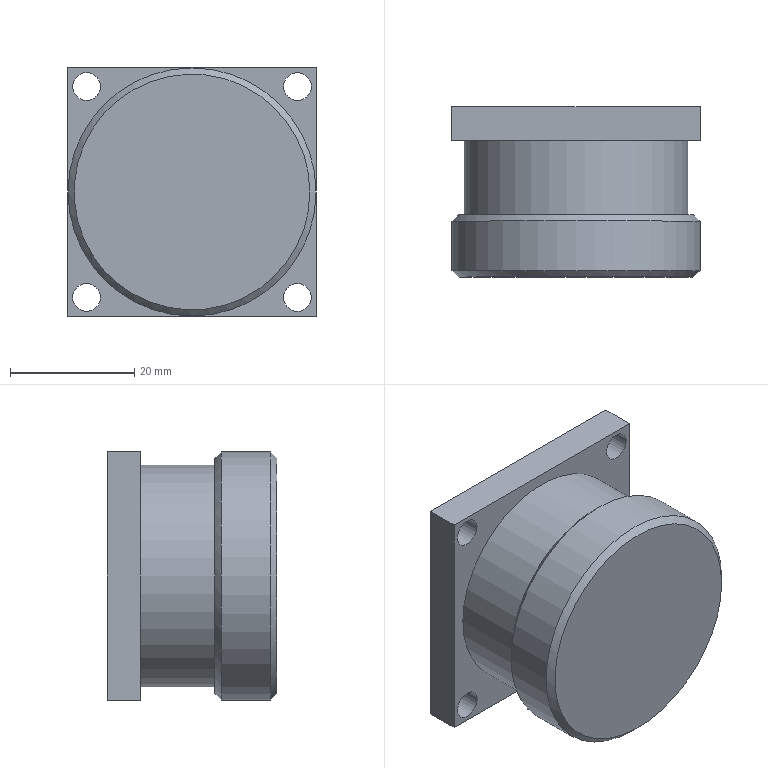Component | NX | BUTTON | 1 solid | 16 faces | box 40 x 27.4 x 40 mm | volume 32954 mm3 | plane 8 | cylinder 6 | cone 2 | commonest cylinder face diameters 4.5 x4 36 x1 40 x1
STEP:
#1=CARTESIAN_POINT('',(0.,0.,0.));
#2=DIRECTION('',(0.,0.,1.));
#3=DIRECTION('',(1.,0.,0.));
#4=AXIS2_PLACEMENT_3D('',#1,#2,#3);
#5=CARTESIAN_POINT('',(-20.,-310.4,-247.));
#6=VERTEX_POINT('',#5);
#7=CARTESIAN_POINT('',(-20.,-310.4,-287.));
#8=VERTEX_POINT('',#7);
#9=CARTESIAN_POINT('',(-20.,-310.4,-247.));
#10=DIRECTION('',(0.,0.,-1.));
#11=VECTOR('',#10,1.);
#12=LINE('',#9,#11);
#13=CARTESIAN_POINT('',(-20.,-305.,-247.));
#14=DIRECTION('',(-1.,0.,0.));
#15=DIRECTION('',(0.,-1.,0.));
#16=AXIS2_PLACEMENT_3D('',#13,#14,#15);
#17=PLANE('',#16);
#18=CARTESIAN_POINT('',(5.4,0.));
#19=DIRECTION('',(0.,-1.));
#20=VECTOR('',#19,1.);
#21=LINE('',#18,#20);
#22=(GEOMETRIC_REPRESENTATION_CONTEXT(2)PARAMETRIC_REPRESENTATION_CONTEXT()REPRESENTATION_CONTEXT('',''));
#23=DEFINITIONAL_REPRESENTATION('',(#21),#22);
#24=PCURVE('',#17,#23);
#25=CARTESIAN_POINT('',(-17.,-310.4,-284.));
#26=DIRECTION('',(0.,-1.,0.));
#27=DIRECTION('',(1.,0.,0.));
#28=AXIS2_PLACEMENT_3D('',#25,#26,#27);
#29=PLANE('',#28);
#30=CARTESIAN_POINT('',(-3.,37.));
#31=DIRECTION('',(0.,-1.));
#32=VECTOR('',#31,1.);
#33=LINE('',#30,#32);
#34=(GEOMETRIC_REPRESENTATION_CONTEXT(2)PARAMETRIC_REPRESENTATION_CONTEXT()REPRESENTATION_CONTEXT('',''));
#35=DEFINITIONAL_REPRESENTATION('',(#33),#34);
#36=PCURVE('',#29,#35);
#37=SURFACE_CURVE('',#12,(#24,#36),.PCURVE_S1.);
#38=EDGE_CURVE('',#6,#8,#37,.T.);
#39=ORIENTED_EDGE('',*,*,#38,.F.);
#40=CARTESIAN_POINT('',(-20.,-305.,-247.));
#41=VERTEX_POINT('',#40);
#42=CARTESIAN_POINT('',(-20.,-305.,-247.));
#43=DIRECTION('',(0.,-1.,0.));
#44=VECTOR('',#43,1.);
#45=LINE('',#42,#44);
#46=CARTESIAN_POINT('',(0.,0.));
#47=DIRECTION('',(1.,0.));
#48=VECTOR('',#47,1.);
#49=LINE('',#46,#48);
#50=(GEOMETRIC_REPRESENTATION_CONTEXT(2)PARAMETRIC_REPRESENTATION_CONTEXT()REPRESENTATION_CONTEXT('',''));
#51=DEFINITIONAL_REPRESENTATION('',(#49),#50);
#52=PCURVE('',#17,#51);
#53=CARTESIAN_POINT('',(20.,-305.,-247.));
#54=DIRECTION('',(0.,0.,1.));
#55=DIRECTION('',(0.,-1.,0.));
#56=AXIS2_PLACEMENT_3D('',#53,#54,#55);
#57=PLANE('',#56);
#58=CARTESIAN_POINT('',(0.,-40.));
#59=DIRECTION('',(1.,0.));
#60=VECTOR('',#59,1.);
#61=LINE('',#58,#60);
#62=(GEOMETRIC_REPRESENTATION_CONTEXT(2)PARAMETRIC_REPRESENTATION_CONTEXT()REPRESENTATION_CONTEXT('',''));
#63=DEFINITIONAL_REPRESENTATION('',(#61),#62);
#64=PCURVE('',#57,#63);
#65=SURFACE_CURVE('',#45,(#52,#64),.PCURVE_S1.);
#66=EDGE_CURVE('',#41,#6,#65,.T.);
#67=ORIENTED_EDGE('',*,*,#66,.F.);
#68=CARTESIAN_POINT('',(-20.,-305.,-287.));
#69=VERTEX_POINT('',#68);
#70=CARTESIAN_POINT('',(-20.,-305.,-247.));
#71=DIRECTION('',(0.,0.,-1.));
#72=VECTOR('',#71,1.);
#73=LINE('',#70,#72);
#74=CARTESIAN_POINT('',(0.,0.));
#75=DIRECTION('',(0.,-1.));
#76=VECTOR('',#75,1.);
#77=LINE('',#74,#76);
#78=(GEOMETRIC_REPRESENTATION_CONTEXT(2)PARAMETRIC_REPRESENTATION_CONTEXT()REPRESENTATION_CONTEXT('',''));
#79=DEFINITIONAL_REPRESENTATION('',(#77),#78);
#80=PCURVE('',#17,#79);
#81=CARTESIAN_POINT('',(-17.,-305.,-284.));
#82=DIRECTION('',(0.,-1.,0.));
#83=DIRECTION('',(1.,0.,0.));
#84=AXIS2_PLACEMENT_3D('',#81,#82,#83);
#85=PLANE('',#84);
#86=CARTESIAN_POINT('',(-3.,37.));
#87=DIRECTION('',(0.,-1.));
#88=VECTOR('',#87,1.);
#89=LINE('',#86,#88);
#90=(GEOMETRIC_REPRESENTATION_CONTEXT(2)PARAMETRIC_REPRESENTATION_CONTEXT()REPRESENTATION_CONTEXT('',''));
#91=DEFINITIONAL_REPRESENTATION('',(#89),#90);
#92=PCURVE('',#85,#91);
#93=SURFACE_CURVE('',#73,(#80,#92),.PCURVE_S1.);
#94=EDGE_CURVE('',#41,#69,#93,.T.);
#95=ORIENTED_EDGE('',*,*,#94,.T.);
#96=CARTESIAN_POINT('',(-20.,-305.,-287.));
#97=DIRECTION('',(0.,-1.,0.));
#98=VECTOR('',#97,1.);
#99=LINE('',#96,#98);
#100=CARTESIAN_POINT('',(0.,-40.));
#101=DIRECTION('',(1.,0.));
#102=VECTOR('',#101,1.);
#103=LINE('',#100,#102);
#104=(GEOMETRIC_REPRESENTATION_CONTEXT(2)PARAMETRIC_REPRESENTATION_CONTEXT()REPRESENTATION_CONTEXT('',''));
#105=DEFINITIONAL_REPRESENTATION('',(#103),#104);
#106=PCURVE('',#17,#105);
#107=CARTESIAN_POINT('',(-20.,-305.,-287.));
#108=DIRECTION('',(0.,0.,-1.));
#109=DIRECTION('',(0.,1.,0.));
#110=AXIS2_PLACEMENT_3D('',#107,#108,#109);
#111=PLANE('',#110);
#112=CARTESIAN_POINT('',(0.,0.));
#113=DIRECTION('',(-1.,0.));
#114=VECTOR('',#113,1.);
#115=LINE('',#112,#114);
#116=(GEOMETRIC_REPRESENTATION_CONTEXT(2)PARAMETRIC_REPRESENTATION_CONTEXT()REPRESENTATION_CONTEXT('',''));
#117=DEFINITIONAL_REPRESENTATION('',(#115),#116);
#118=PCURVE('',#111,#117);
#119=SURFACE_CURVE('',#99,(#106,#118),.PCURVE_S1.);
#120=EDGE_CURVE('',#69,#8,#119,.T.);
#121=ORIENTED_EDGE('',*,*,#120,.T.);
#122=EDGE_LOOP('',(#39,#67,#95,#121));
#123=FACE_BOUND('',#122,.T.);
#124=ADVANCED_FACE('',(#123),#17,.T.);
#125=CARTESIAN_POINT('',(20.,-310.4,-287.));
#126=VERTEX_POINT('',#125);
#127=CARTESIAN_POINT('',(-20.,-310.4,-287.));
#128=DIRECTION('',(1.,0.,0.));
#129=VECTOR('',#128,1.);
#130=LINE('',#127,#129);
#131=CARTESIAN_POINT('',(-5.4,0.));
#132=DIRECTION('',(0.,1.));
#133=VECTOR('',#132,1.);
#134=LINE('',#131,#133);
#135=(GEOMETRIC_REPRESENTATION_CONTEXT(2)PARAMETRIC_REPRESENTATION_CONTEXT()REPRESENTATION_CONTEXT('',''));
#136=DEFINITIONAL_REPRESENTATION('',(#134),#135);
#137=PCURVE('',#111,#136);
#138=CARTESIAN_POINT('',(-3.,-3.));
#139=DIRECTION('',(1.,0.));
#140=VECTOR('',#139,1.);
#141=LINE('',#138,#140);
#142=(GEOMETRIC_REPRESENTATION_CONTEXT(2)PARAMETRIC_REPRESENTATION_CONTEXT()REPRESENTATION_CONTEXT('',''));
#143=DEFINITIONAL_REPRESENTATION('',(#141),#142);
#144=PCURVE('',#29,#143);
#145=SURFACE_CURVE('',#130,(#137,#144),.PCURVE_S1.);
#146=EDGE_CURVE('',#8,#126,#145,.T.);
#147=ORIENTED_EDGE('',*,*,#146,.F.);
#148=ORIENTED_EDGE('',*,*,#120,.F.);
#149=CARTESIAN_POINT('',(20.,-305.,-287.));
#150=VERTEX_POINT('',#149);
#151=CARTESIAN_POINT('',(-20.,-305.,-287.));
#152=DIRECTION('',(1.,0.,0.));
#153=VECTOR('',#152,1.);
#154=LINE('',#151,#153);
#155=CARTESIAN_POINT('',(0.,0.));
#156=DIRECTION('',(0.,1.));
#157=VECTOR('',#156,1.);
#158=LINE('',#155,#157);
#159=(GEOMETRIC_REPRESENTATION_CONTEXT(2)PARAMETRIC_REPRESENTATION_CONTEXT()REPRESENTATION_CONTEXT('',''));
#160=DEFINITIONAL_REPRESENTATION('',(#158),#159);
#161=PCURVE('',#111,#160);
#162=CARTESIAN_POINT('',(-3.,-3.));
#163=DIRECTION('',(1.,0.));
#164=VECTOR('',#163,1.);
#165=LINE('',#162,#164);
#166=(GEOMETRIC_REPRESENTATION_CONTEXT(2)PARAMETRIC_REPRESENTATION_CONTEXT()REPRESENTATION_CONTEXT('',''));
#167=DEFINITIONAL_REPRESENTATION('',(#165),#166);
#168=PCURVE('',#85,#167);
#169=SURFACE_CURVE('',#154,(#161,#168),.PCURVE_S1.);
#170=EDGE_CURVE('',#69,#150,#169,.T.);
#171=ORIENTED_EDGE('',*,*,#170,.T.);
#172=CARTESIAN_POINT('',(20.,-305.,-287.));
#173=DIRECTION('',(0.,-1.,0.));
#174=VECTOR('',#173,1.);
#175=LINE('',#172,#174);
#176=CARTESIAN_POINT('',(0.,40.));
#177=DIRECTION('',(-1.,0.));
#178=VECTOR('',#177,1.);
#179=LINE('',#176,#178);
#180=(GEOMETRIC_REPRESENTATION_CONTEXT(2)PARAMETRIC_REPRESENTATION_CONTEXT()REPRESENTATION_CONTEXT('',''));
#181=DEFINITIONAL_REPRESENTATION('',(#179),#180);
#182=PCURVE('',#111,#181);
#183=CARTESIAN_POINT('',(20.,-305.,-287.));
#184=DIRECTION('',(1.,0.,0.));
#185=DIRECTION('',(0.,1.,0.));
#186=AXIS2_PLACEMENT_3D('',#183,#184,#185);
#187=PLANE('',#186);
#188=CARTESIAN_POINT('',(0.,0.));
#189=DIRECTION('',(-1.,0.));
#190=VECTOR('',#189,1.);
#191=LINE('',#188,#190);
#192=(GEOMETRIC_REPRESENTATION_CONTEXT(2)PARAMETRIC_REPRESENTATION_CONTEXT()REPRESENTATION_CONTEXT('',''));
#193=DEFINITIONAL_REPRESENTATION('',(#191),#192);
#194=PCURVE('',#187,#193);
#195=SURFACE_CURVE('',#175,(#182,#194),.PCURVE_S1.);
#196=EDGE_CURVE('',#150,#126,#195,.T.);
#197=ORIENTED_EDGE('',*,*,#196,.T.);
#198=EDGE_LOOP('',(#147,#148,#171,#197));
#199=FACE_BOUND('',#198,.T.);
#200=ADVANCED_FACE('',(#199),#111,.T.);
#201=CARTESIAN_POINT('',(20.,-310.4,-247.));
#202=VERTEX_POINT('',#201);
#203=CARTESIAN_POINT('',(20.,-310.4,-287.));
#204=DIRECTION('',(0.,0.,1.));
#205=VECTOR('',#204,1.);
#206=LINE('',#203,#205);
#207=CARTESIAN_POINT('',(-5.4,0.));
#208=DIRECTION('',(0.,1.));
#209=VECTOR('',#208,1.);
#210=LINE('',#207,#209);
#211=(GEOMETRIC_REPRESENTATION_CONTEXT(2)PARAMETRIC_REPRESENTATION_CONTEXT()REPRESENTATION_CONTEXT('',''));
#212=DEFINITIONAL_REPRESENTATION('',(#210),#211);
#213=PCURVE('',#187,#212);
#214=CARTESIAN_POINT('',(37.,-3.));
#215=DIRECTION('',(0.,1.));
#216=VECTOR('',#215,1.);
#217=LINE('',#214,#216);
#218=(GEOMETRIC_REPRESENTATION_CONTEXT(2)PARAMETRIC_REPRESENTATION_CONTEXT()REPRESENTATION_CONTEXT('',''));
#219=DEFINITIONAL_REPRESENTATION('',(#217),#218);
#220=PCURVE('',#29,#219);
#221=SURFACE_CURVE('',#206,(#213,#220),.PCURVE_S1.);
#222=EDGE_CURVE('',#126,#202,#221,.T.);
#223=ORIENTED_EDGE('',*,*,#222,.F.);
#224=ORIENTED_EDGE('',*,*,#196,.F.);
#225=CARTESIAN_POINT('',(20.,-305.,-247.));
#226=VERTEX_POINT('',#225);
#227=CARTESIAN_POINT('',(20.,-305.,-287.));
#228=DIRECTION('',(0.,0.,1.));
#229=VECTOR('',#228,1.);
#230=LINE('',#227,#229);
#231=CARTESIAN_POINT('',(0.,0.));
#232=DIRECTION('',(0.,1.));
#233=VECTOR('',#232,1.);
#234=LINE('',#231,#233);
#235=(GEOMETRIC_REPRESENTATION_CONTEXT(2)PARAMETRIC_REPRESENTATION_CONTEXT()REPRESENTATION_CONTEXT('',''));
#236=DEFINITIONAL_REPRESENTATION('',(#234),#235);
#237=PCURVE('',#187,#236);
#238=CARTESIAN_POINT('',(37.,-3.));
#239=DIRECTION('',(0.,1.));
#240=VECTOR('',#239,1.);
#241=LINE('',#238,#240);
#242=(GEOMETRIC_REPRESENTATION_CONTEXT(2)PARAMETRIC_REPRESENTATION_CONTEXT()REPRESENTATION_CONTEXT('',''));
#243=DEFINITIONAL_REPRESENTATION('',(#241),#242);
#244=PCURVE('',#85,#243);
#245=SURFACE_CURVE('',#230,(#237,#244),.PCURVE_S1.);
#246=EDGE_CURVE('',#150,#226,#245,.T.);
#247=ORIENTED_EDGE('',*,*,#246,.T.);
#248=CARTESIAN_POINT('',(20.,-305.,-247.));
#249=DIRECTION('',(0.,-1.,0.));
#250=VECTOR('',#249,1.);
#251=LINE('',#248,#250);
#252=CARTESIAN_POINT('',(0.,40.));
#253=DIRECTION('',(-1.,0.));
#254=VECTOR('',#253,1.);
#255=LINE('',#252,#254);
#256=(GEOMETRIC_REPRESENTATION_CONTEXT(2)PARAMETRIC_REPRESENTATION_CONTEXT()REPRESENTATION_CONTEXT('',''));
#257=DEFINITIONAL_REPRESENTATION('',(#255),#256);
#258=PCURVE('',#187,#257);
#259=CARTESIAN_POINT('',(0.,0.));
#260=DIRECTION('',(1.,0.));
#261=VECTOR('',#260,1.);
#262=LINE('',#259,#261);
#263=(GEOMETRIC_REPRESENTATION_CONTEXT(2)PARAMETRIC_REPRESENTATION_CONTEXT()REPRESENTATION_CONTEXT('',''));
#264=DEFINITIONAL_REPRESENTATION('',(#262),#263);
#265=PCURVE('',#57,#264);
#266=SURFACE_CURVE('',#251,(#258,#265),.PCURVE_S1.);
#267=EDGE_CURVE('',#226,#202,#266,.T.);
#268=ORIENTED_EDGE('',*,*,#267,.T.);
#269=EDGE_LOOP('',(#223,#224,#247,#268));
#270=FACE_BOUND('',#269,.T.);
#271=ADVANCED_FACE('',(#270),#187,.T.);
#272=CARTESIAN_POINT('',(14.75,-305.,-284.));
#273=VERTEX_POINT('',#272);
#274=CARTESIAN_POINT('',(17.,-305.,-284.));
#275=DIRECTION('',(0.,-1.,0.));
#276=DIRECTION('',(-1.,0.,0.));
#277=AXIS2_PLACEMENT_3D('',#274,#275,#276);
#278=CIRCLE('',#277,2.25);
#279=CARTESIAN_POINT('',(17.,-305.,-284.));
#280=DIRECTION('',(0.,-1.,0.));
#281=DIRECTION('',(1.,0.,0.));
#282=AXIS2_PLACEMENT_3D('',#279,#280,#281);
#283=CYLINDRICAL_SURFACE('',#282,2.25);
#284=CARTESIAN_POINT('',(3.142,0.));
#285=DIRECTION('',(1.,0.));
#286=VECTOR('',#285,1.);
#287=LINE('',#284,#286);
#288=(GEOMETRIC_REPRESENTATION_CONTEXT(2)PARAMETRIC_REPRESENTATION_CONTEXT()REPRESENTATION_CONTEXT('',''));
#289=DEFINITIONAL_REPRESENTATION('',(#287),#288);
#290=PCURVE('',#283,#289);
#291=CARTESIAN_POINT('',(34.,0.));
#292=DIRECTION('',(-1.,0.));
#293=AXIS2_PLACEMENT_2D('',#291,#292);
#294=CIRCLE('',#293,2.25);
#295=(GEOMETRIC_REPRESENTATION_CONTEXT(2)PARAMETRIC_REPRESENTATION_CONTEXT()REPRESENTATION_CONTEXT('',''));
#296=DEFINITIONAL_REPRESENTATION('',(#294),#295);
#297=PCURVE('',#85,#296);
#298=SURFACE_CURVE('',#278,(#290,#297),.PCURVE_S1.);
#299=EDGE_CURVE('',#273,#273,#298,.T.);
#300=ORIENTED_EDGE('',*,*,#299,.T.);
#301=CARTESIAN_POINT('',(14.75,-310.4,-284.));
#302=VERTEX_POINT('',#301);
#303=CARTESIAN_POINT('',(14.75,-305.,-284.));
#304=CARTESIAN_POINT('',(14.75,-310.4,-284.));
#305=B_SPLINE_CURVE_WITH_KNOTS('',1,(#303,#304),.UNSPECIFIED.,.F.,.F.,(2,2),(0.,5.4),.PIECEWISE_BEZIER_KNOTS.);
#306=CARTESIAN_POINT('',(9.425,0.));
#307=DIRECTION('',(0.,1.));
#308=VECTOR('',#307,1.);
#309=LINE('',#306,#308);
#310=(GEOMETRIC_REPRESENTATION_CONTEXT(2)PARAMETRIC_REPRESENTATION_CONTEXT()REPRESENTATION_CONTEXT('',''));
#311=DEFINITIONAL_REPRESENTATION('',(#309),#310);
#312=PCURVE('',#283,#311);
#313=CARTESIAN_POINT('',(3.142,0.));
#314=DIRECTION('',(0.,1.));
#315=VECTOR('',#314,1.);
#316=LINE('',#313,#315);
#317=(GEOMETRIC_REPRESENTATION_CONTEXT(2)PARAMETRIC_REPRESENTATION_CONTEXT()REPRESENTATION_CONTEXT('',''));
#318=DEFINITIONAL_REPRESENTATION('',(#316),#317);
#319=PCURVE('',#283,#318);
#320=SEAM_CURVE('',#305,(#312,#319),.PCURVE_S1.);
#321=EDGE_CURVE('',#273,#302,#320,.T.);
#322=ORIENTED_EDGE('',*,*,#321,.T.);
#323=CARTESIAN_POINT('',(17.,-310.4,-284.));
#324=DIRECTION('',(0.,-1.,0.));
#325=DIRECTION('',(-1.,0.,0.));
#326=AXIS2_PLACEMENT_3D('',#323,#324,#325);
#327=CIRCLE('',#326,2.25);
#328=CARTESIAN_POINT('',(3.142,5.4));
#329=DIRECTION('',(1.,0.));
#330=VECTOR('',#329,1.);
#331=LINE('',#328,#330);
#332=(GEOMETRIC_REPRESENTATION_CONTEXT(2)PARAMETRIC_REPRESENTATION_CONTEXT()REPRESENTATION_CONTEXT('',''));
#333=DEFINITIONAL_REPRESENTATION('',(#331),#332);
#334=PCURVE('',#283,#333);
#335=CARTESIAN_POINT('',(34.,0.));
#336=DIRECTION('',(-1.,0.));
#337=AXIS2_PLACEMENT_2D('',#335,#336);
#338=CIRCLE('',#337,2.25);
#339=(GEOMETRIC_REPRESENTATION_CONTEXT(2)PARAMETRIC_REPRESENTATION_CONTEXT()REPRESENTATION_CONTEXT('',''));
#340=DEFINITIONAL_REPRESENTATION('',(#338),#339);
#341=PCURVE('',#29,#340);
#342=SURFACE_CURVE('',#327,(#334,#341),.PCURVE_S1.);
#343=EDGE_CURVE('',#302,#302,#342,.T.);
#344=ORIENTED_EDGE('',*,*,#343,.F.);
#345=ORIENTED_EDGE('',*,*,#321,.F.);
#346=EDGE_LOOP('',(#300,#322,#344,#345));
#347=FACE_BOUND('',#346,.F.);
#348=ADVANCED_FACE('',(#347),#283,.F.);
#349=CARTESIAN_POINT('',(-14.75,-305.,-250.));
#350=VERTEX_POINT('',#349);
#351=CARTESIAN_POINT('',(-17.,-305.,-250.));
#352=DIRECTION('',(0.,-1.,0.));
#353=DIRECTION('',(1.,0.,0.));
#354=AXIS2_PLACEMENT_3D('',#351,#352,#353);
#355=CIRCLE('',#354,2.25);
#356=CARTESIAN_POINT('',(-17.,-305.,-250.));
#357=DIRECTION('',(0.,-1.,0.));
#358=DIRECTION('',(1.,0.,0.));
#359=AXIS2_PLACEMENT_3D('',#356,#357,#358);
#360=CYLINDRICAL_SURFACE('',#359,2.25);
#361=CARTESIAN_POINT('',(0.,0.));
#362=DIRECTION('',(1.,0.));
#363=VECTOR('',#362,1.);
#364=LINE('',#361,#363);
#365=(GEOMETRIC_REPRESENTATION_CONTEXT(2)PARAMETRIC_REPRESENTATION_CONTEXT()REPRESENTATION_CONTEXT('',''));
#366=DEFINITIONAL_REPRESENTATION('',(#364),#365);
#367=PCURVE('',#360,#366);
#368=CARTESIAN_POINT('',(0.,34.));
#369=DIRECTION('',(1.,0.));
#370=AXIS2_PLACEMENT_2D('',#368,#369);
#371=CIRCLE('',#370,2.25);
#372=(GEOMETRIC_REPRESENTATION_CONTEXT(2)PARAMETRIC_REPRESENTATION_CONTEXT()REPRESENTATION_CONTEXT('',''));
#373=DEFINITIONAL_REPRESENTATION('',(#371),#372);
#374=PCURVE('',#85,#373);
#375=SURFACE_CURVE('',#355,(#367,#374),.PCURVE_S1.);
#376=EDGE_CURVE('',#350,#350,#375,.T.);
#377=ORIENTED_EDGE('',*,*,#376,.T.);
#378=CARTESIAN_POINT('',(-14.75,-310.4,-250.));
#379=VERTEX_POINT('',#378);
#380=CARTESIAN_POINT('',(-14.75,-305.,-250.));
#381=CARTESIAN_POINT('',(-14.75,-310.4,-250.));
#382=B_SPLINE_CURVE_WITH_KNOTS('',1,(#380,#381),.UNSPECIFIED.,.F.,.F.,(2,2),(0.,5.4),.PIECEWISE_BEZIER_KNOTS.);
#383=CARTESIAN_POINT('',(6.283,0.));
#384=DIRECTION('',(0.,1.));
#385=VECTOR('',#384,1.);
#386=LINE('',#383,#385);
#387=(GEOMETRIC_REPRESENTATION_CONTEXT(2)PARAMETRIC_REPRESENTATION_CONTEXT()REPRESENTATION_CONTEXT('',''));
#388=DEFINITIONAL_REPRESENTATION('',(#386),#387);
#389=PCURVE('',#360,#388);
#390=CARTESIAN_POINT('',(0.,0.));
#391=DIRECTION('',(0.,1.));
#392=VECTOR('',#391,1.);
#393=LINE('',#390,#392);
#394=(GEOMETRIC_REPRESENTATION_CONTEXT(2)PARAMETRIC_REPRESENTATION_CONTEXT()REPRESENTATION_CONTEXT('',''));
#395=DEFINITIONAL_REPRESENTATION('',(#393),#394);
#396=PCURVE('',#360,#395);
#397=SEAM_CURVE('',#382,(#389,#396),.PCURVE_S1.);
#398=EDGE_CURVE('',#350,#379,#397,.T.);
#399=ORIENTED_EDGE('',*,*,#398,.T.);
#400=CARTESIAN_POINT('',(-17.,-310.4,-250.));
#401=DIRECTION('',(0.,-1.,0.));
#402=DIRECTION('',(1.,0.,0.));
#403=AXIS2_PLACEMENT_3D('',#400,#401,#402);
#404=CIRCLE('',#403,2.25);
#405=CARTESIAN_POINT('',(0.,5.4));
#406=DIRECTION('',(1.,0.));
#407=VECTOR('',#406,1.);
#408=LINE('',#405,#407);
#409=(GEOMETRIC_REPRESENTATION_CONTEXT(2)PARAMETRIC_REPRESENTATION_CONTEXT()REPRESENTATION_CONTEXT('',''));
#410=DEFINITIONAL_REPRESENTATION('',(#408),#409);
#411=PCURVE('',#360,#410);
#412=CARTESIAN_POINT('',(0.,34.));
#413=DIRECTION('',(1.,0.));
#414=AXIS2_PLACEMENT_2D('',#412,#413);
#415=CIRCLE('',#414,2.25);
#416=(GEOMETRIC_REPRESENTATION_CONTEXT(2)PARAMETRIC_REPRESENTATION_CONTEXT()REPRESENTATION_CONTEXT('',''));
#417=DEFINITIONAL_REPRESENTATION('',(#415),#416);
#418=PCURVE('',#29,#417);
#419=SURFACE_CURVE('',#404,(#411,#418),.PCURVE_S1.);
#420=EDGE_CURVE('',#379,#379,#419,.T.);
#421=ORIENTED_EDGE('',*,*,#420,.F.);
#422=ORIENTED_EDGE('',*,*,#398,.F.);
#423=EDGE_LOOP('',(#377,#399,#421,#422));
#424=FACE_BOUND('',#423,.F.);
#425=ADVANCED_FACE('',(#424),#360,.F.);
#426=CARTESIAN_POINT('',(-17.,-305.,-281.75));
#427=VERTEX_POINT('',#426);
#428=CARTESIAN_POINT('',(-17.,-305.,-284.));
#429=DIRECTION('',(0.,-1.,0.));
#430=DIRECTION('',(0.,0.,1.));
#431=AXIS2_PLACEMENT_3D('',#428,#429,#430);
#432=CIRCLE('',#431,2.25);
#433=CARTESIAN_POINT('',(-17.,-305.,-284.));
#434=DIRECTION('',(0.,-1.,0.));
#435=DIRECTION('',(1.,0.,0.));
#436=AXIS2_PLACEMENT_3D('',#433,#434,#435);
#437=CYLINDRICAL_SURFACE('',#436,2.25);
#438=CARTESIAN_POINT('',(1.571,0.));
#439=DIRECTION('',(1.,0.));
#440=VECTOR('',#439,1.);
#441=LINE('',#438,#440);
#442=(GEOMETRIC_REPRESENTATION_CONTEXT(2)PARAMETRIC_REPRESENTATION_CONTEXT()REPRESENTATION_CONTEXT('',''));
#443=DEFINITIONAL_REPRESENTATION('',(#441),#442);
#444=PCURVE('',#437,#443);
#445=CARTESIAN_POINT('',(0.,0.));
#446=DIRECTION('',(0.,1.));
#447=AXIS2_PLACEMENT_2D('',#445,#446);
#448=CIRCLE('',#447,2.25);
#449=(GEOMETRIC_REPRESENTATION_CONTEXT(2)PARAMETRIC_REPRESENTATION_CONTEXT()REPRESENTATION_CONTEXT('',''));
#450=DEFINITIONAL_REPRESENTATION('',(#448),#449);
#451=PCURVE('',#85,#450);
#452=SURFACE_CURVE('',#432,(#444,#451),.PCURVE_S1.);
#453=EDGE_CURVE('',#427,#427,#452,.T.);
#454=ORIENTED_EDGE('',*,*,#453,.T.);
#455=CARTESIAN_POINT('',(-17.,-310.4,-281.75));
#456=VERTEX_POINT('',#455);
#457=CARTESIAN_POINT('',(-17.,-305.,-281.75));
#458=CARTESIAN_POINT('',(-17.,-310.4,-281.75));
#459=B_SPLINE_CURVE_WITH_KNOTS('',1,(#457,#458),.UNSPECIFIED.,.F.,.F.,(2,2),(0.,5.4),.PIECEWISE_BEZIER_KNOTS.);
#460=CARTESIAN_POINT('',(7.854,0.));
#461=DIRECTION('',(0.,1.));
#462=VECTOR('',#461,1.);
#463=LINE('',#460,#462);
#464=(GEOMETRIC_REPRESENTATION_CONTEXT(2)PARAMETRIC_REPRESENTATION_CONTEXT()REPRESENTATION_CONTEXT('',''));
#465=DEFINITIONAL_REPRESENTATION('',(#463),#464);
#466=PCURVE('',#437,#465);
#467=CARTESIAN_POINT('',(1.571,0.));
#468=DIRECTION('',(0.,1.));
#469=VECTOR('',#468,1.);
#470=LINE('',#467,#469);
#471=(GEOMETRIC_REPRESENTATION_CONTEXT(2)PARAMETRIC_REPRESENTATION_CONTEXT()REPRESENTATION_CONTEXT('',''));
#472=DEFINITIONAL_REPRESENTATION('',(#470),#471);
#473=PCURVE('',#437,#472);
#474=SEAM_CURVE('',#459,(#466,#473),.PCURVE_S1.);
#475=EDGE_CURVE('',#427,#456,#474,.T.);
#476=ORIENTED_EDGE('',*,*,#475,.T.);
#477=CARTESIAN_POINT('',(-17.,-310.4,-284.));
#478=DIRECTION('',(0.,-1.,0.));
#479=DIRECTION('',(0.,0.,1.));
#480=AXIS2_PLACEMENT_3D('',#477,#478,#479);
#481=CIRCLE('',#480,2.25);
#482=CARTESIAN_POINT('',(1.571,5.4));
#483=DIRECTION('',(1.,0.));
#484=VECTOR('',#483,1.);
#485=LINE('',#482,#484);
#486=(GEOMETRIC_REPRESENTATION_CONTEXT(2)PARAMETRIC_REPRESENTATION_CONTEXT()REPRESENTATION_CONTEXT('',''));
#487=DEFINITIONAL_REPRESENTATION('',(#485),#486);
#488=PCURVE('',#437,#487);
#489=CARTESIAN_POINT('',(0.,0.));
#490=DIRECTION('',(0.,1.));
#491=AXIS2_PLACEMENT_2D('',#489,#490);
#492=CIRCLE('',#491,2.25);
#493=(GEOMETRIC_REPRESENTATION_CONTEXT(2)PARAMETRIC_REPRESENTATION_CONTEXT()REPRESENTATION_CONTEXT('',''));
#494=DEFINITIONAL_REPRESENTATION('',(#492),#493);
#495=PCURVE('',#29,#494);
#496=SURFACE_CURVE('',#481,(#488,#495),.PCURVE_S1.);
#497=EDGE_CURVE('',#456,#456,#496,.T.);
#498=ORIENTED_EDGE('',*,*,#497,.F.);
#499=ORIENTED_EDGE('',*,*,#475,.F.);
#500=EDGE_LOOP('',(#454,#476,#498,#499));
#501=FACE_BOUND('',#500,.F.);
#502=ADVANCED_FACE('',(#501),#437,.F.);
#503=CARTESIAN_POINT('',(20.,-310.4,-247.));
#504=DIRECTION('',(-1.,0.,0.));
#505=VECTOR('',#504,1.);
#506=LINE('',#503,#505);
#507=CARTESIAN_POINT('',(5.4,0.));
#508=DIRECTION('',(0.,-1.));
#509=VECTOR('',#508,1.);
#510=LINE('',#507,#509);
#511=(GEOMETRIC_REPRESENTATION_CONTEXT(2)PARAMETRIC_REPRESENTATION_CONTEXT()REPRESENTATION_CONTEXT('',''));
#512=DEFINITIONAL_REPRESENTATION('',(#510),#511);
#513=PCURVE('',#57,#512);
#514=CARTESIAN_POINT('',(37.,37.));
#515=DIRECTION('',(-1.,0.));
#516=VECTOR('',#515,1.);
#517=LINE('',#514,#516);
#518=(GEOMETRIC_REPRESENTATION_CONTEXT(2)PARAMETRIC_REPRESENTATION_CONTEXT()REPRESENTATION_CONTEXT('',''));
#519=DEFINITIONAL_REPRESENTATION('',(#517),#518);
#520=PCURVE('',#29,#519);
#521=SURFACE_CURVE('',#506,(#513,#520),.PCURVE_S1.);
#522=EDGE_CURVE('',#202,#6,#521,.T.);
#523=ORIENTED_EDGE('',*,*,#522,.F.);
#524=ORIENTED_EDGE('',*,*,#267,.F.);
#525=CARTESIAN_POINT('',(20.,-305.,-247.));
#526=DIRECTION('',(-1.,0.,0.));
#527=VECTOR('',#526,1.);
#528=LINE('',#525,#527);
#529=CARTESIAN_POINT('',(0.,0.));
#530=DIRECTION('',(0.,-1.));
#531=VECTOR('',#530,1.);
#532=LINE('',#529,#531);
#533=(GEOMETRIC_REPRESENTATION_CONTEXT(2)PARAMETRIC_REPRESENTATION_CONTEXT()REPRESENTATION_CONTEXT('',''));
#534=DEFINITIONAL_REPRESENTATION('',(#532),#533);
#535=PCURVE('',#57,#534);
#536=CARTESIAN_POINT('',(37.,37.));
#537=DIRECTION('',(-1.,0.));
#538=VECTOR('',#537,1.);
#539=LINE('',#536,#538);
#540=(GEOMETRIC_REPRESENTATION_CONTEXT(2)PARAMETRIC_REPRESENTATION_CONTEXT()REPRESENTATION_CONTEXT('',''));
#541=DEFINITIONAL_REPRESENTATION('',(#539),#540);
#542=PCURVE('',#85,#541);
#543=SURFACE_CURVE('',#528,(#535,#542),.PCURVE_S1.);
#544=EDGE_CURVE('',#226,#41,#543,.T.);
#545=ORIENTED_EDGE('',*,*,#544,.T.);
#546=ORIENTED_EDGE('',*,*,#66,.T.);
#547=EDGE_LOOP('',(#523,#524,#545,#546));
#548=FACE_BOUND('',#547,.T.);
#549=ADVANCED_FACE('',(#548),#57,.T.);
#550=CARTESIAN_POINT('',(17.,-305.,-252.25));
#551=VERTEX_POINT('',#550);
#552=CARTESIAN_POINT('',(17.,-305.,-250.));
#553=DIRECTION('',(0.,-1.,0.));
#554=DIRECTION('',(0.,0.,-1.));
#555=AXIS2_PLACEMENT_3D('',#552,#553,#554);
#556=CIRCLE('',#555,2.25);
#557=CARTESIAN_POINT('',(17.,-305.,-250.));
#558=DIRECTION('',(0.,-1.,0.));
#559=DIRECTION('',(1.,0.,0.));
#560=AXIS2_PLACEMENT_3D('',#557,#558,#559);
#561=CYLINDRICAL_SURFACE('',#560,2.25);
#562=CARTESIAN_POINT('',(4.712,0.));
#563=DIRECTION('',(1.,0.));
#564=VECTOR('',#563,1.);
#565=LINE('',#562,#564);
#566=(GEOMETRIC_REPRESENTATION_CONTEXT(2)PARAMETRIC_REPRESENTATION_CONTEXT()REPRESENTATION_CONTEXT('',''));
#567=DEFINITIONAL_REPRESENTATION('',(#565),#566);
#568=PCURVE('',#561,#567);
#569=CARTESIAN_POINT('',(34.,34.));
#570=DIRECTION('',(0.,-1.));
#571=AXIS2_PLACEMENT_2D('',#569,#570);
#572=CIRCLE('',#571,2.25);
#573=(GEOMETRIC_REPRESENTATION_CONTEXT(2)PARAMETRIC_REPRESENTATION_CONTEXT()REPRESENTATION_CONTEXT('',''));
#574=DEFINITIONAL_REPRESENTATION('',(#572),#573);
#575=PCURVE('',#85,#574);
#576=SURFACE_CURVE('',#556,(#568,#575),.PCURVE_S1.);
#577=EDGE_CURVE('',#551,#551,#576,.T.);
#578=ORIENTED_EDGE('',*,*,#577,.T.);
#579=CARTESIAN_POINT('',(17.,-310.4,-252.25));
#580=VERTEX_POINT('',#579);
#581=CARTESIAN_POINT('',(17.,-305.,-252.25));
#582=CARTESIAN_POINT('',(17.,-310.4,-252.25));
#583=B_SPLINE_CURVE_WITH_KNOTS('',1,(#581,#582),.UNSPECIFIED.,.F.,.F.,(2,2),(0.,5.4),.PIECEWISE_BEZIER_KNOTS.);
#584=CARTESIAN_POINT('',(10.996,0.));
#585=DIRECTION('',(0.,1.));
#586=VECTOR('',#585,1.);
#587=LINE('',#584,#586);
#588=(GEOMETRIC_REPRESENTATION_CONTEXT(2)PARAMETRIC_REPRESENTATION_CONTEXT()REPRESENTATION_CONTEXT('',''));
#589=DEFINITIONAL_REPRESENTATION('',(#587),#588);
#590=PCURVE('',#561,#589);
#591=CARTESIAN_POINT('',(4.712,0.));
#592=DIRECTION('',(0.,1.));
#593=VECTOR('',#592,1.);
#594=LINE('',#591,#593);
#595=(GEOMETRIC_REPRESENTATION_CONTEXT(2)PARAMETRIC_REPRESENTATION_CONTEXT()REPRESENTATION_CONTEXT('',''));
#596=DEFINITIONAL_REPRESENTATION('',(#594),#595);
#597=PCURVE('',#561,#596);
#598=SEAM_CURVE('',#583,(#590,#597),.PCURVE_S1.);
#599=EDGE_CURVE('',#551,#580,#598,.T.);
#600=ORIENTED_EDGE('',*,*,#599,.T.);
#601=CARTESIAN_POINT('',(17.,-310.4,-250.));
#602=DIRECTION('',(0.,-1.,0.));
#603=DIRECTION('',(0.,0.,-1.));
#604=AXIS2_PLACEMENT_3D('',#601,#602,#603);
#605=CIRCLE('',#604,2.25);
#606=CARTESIAN_POINT('',(4.712,5.4));
#607=DIRECTION('',(1.,0.));
#608=VECTOR('',#607,1.);
#609=LINE('',#606,#608);
#610=(GEOMETRIC_REPRESENTATION_CONTEXT(2)PARAMETRIC_REPRESENTATION_CONTEXT()REPRESENTATION_CONTEXT('',''));
#611=DEFINITIONAL_REPRESENTATION('',(#609),#610);
#612=PCURVE('',#561,#611);
#613=CARTESIAN_POINT('',(34.,34.));
#614=DIRECTION('',(0.,-1.));
#615=AXIS2_PLACEMENT_2D('',#613,#614);
#616=CIRCLE('',#615,2.25);
#617=(GEOMETRIC_REPRESENTATION_CONTEXT(2)PARAMETRIC_REPRESENTATION_CONTEXT()REPRESENTATION_CONTEXT('',''));
#618=DEFINITIONAL_REPRESENTATION('',(#616),#617);
#619=PCURVE('',#29,#618);
#620=SURFACE_CURVE('',#605,(#612,#619),.PCURVE_S1.);
#621=EDGE_CURVE('',#580,#580,#620,.T.);
#622=ORIENTED_EDGE('',*,*,#621,.F.);
#623=ORIENTED_EDGE('',*,*,#599,.F.);
#624=EDGE_LOOP('',(#578,#600,#622,#623));
#625=FACE_BOUND('',#624,.F.);
#626=ADVANCED_FACE('',(#625),#561,.F.);
#627=ORIENTED_EDGE('',*,*,#94,.F.);
#628=ORIENTED_EDGE('',*,*,#544,.F.);
#629=ORIENTED_EDGE('',*,*,#246,.F.);
#630=ORIENTED_EDGE('',*,*,#170,.F.);
#631=EDGE_LOOP('',(#627,#628,#629,#630));
#632=FACE_BOUND('',#631,.T.);
#633=ORIENTED_EDGE('',*,*,#453,.T.);
#634=EDGE_LOOP('',(#633));
#635=FACE_BOUND('',#634,.T.);
#636=ORIENTED_EDGE('',*,*,#376,.T.);
#637=EDGE_LOOP('',(#636));
#638=FACE_BOUND('',#637,.T.);
#639=ORIENTED_EDGE('',*,*,#299,.T.);
#640=EDGE_LOOP('',(#639));
#641=FACE_BOUND('',#640,.T.);
#642=ORIENTED_EDGE('',*,*,#577,.T.);
#643=EDGE_LOOP('',(#642));
#644=FACE_BOUND('',#643,.T.);
#645=ADVANCED_FACE('',(#632,#635,#638,#641,#644),#85,.F.);
#646=CARTESIAN_POINT('',(18.,-310.4,-267.));
#647=VERTEX_POINT('',#646);
#648=CARTESIAN_POINT('',(-0.,-310.4,-267.));
#649=DIRECTION('',(0.,-1.,0.));
#650=DIRECTION('',(1.,0.,0.));
#651=AXIS2_PLACEMENT_3D('',#648,#649,#650);
#652=CIRCLE('',#651,18.);
#653=CARTESIAN_POINT('',(17.,17.));
#654=DIRECTION('',(1.,0.));
#655=AXIS2_PLACEMENT_2D('',#653,#654);
#656=CIRCLE('',#655,18.);
#657=(GEOMETRIC_REPRESENTATION_CONTEXT(2)PARAMETRIC_REPRESENTATION_CONTEXT()REPRESENTATION_CONTEXT('',''));
#658=DEFINITIONAL_REPRESENTATION('',(#656),#657);
#659=PCURVE('',#29,#658);
#660=CARTESIAN_POINT('',(-0.,-322.4,-267.));
#661=DIRECTION('',(0.,1.,0.));
#662=DIRECTION('',(-1.,0.,0.));
#663=AXIS2_PLACEMENT_3D('',#660,#661,#662);
#664=CYLINDRICAL_SURFACE('',#663,18.);
#665=CARTESIAN_POINT('',(9.425,12.));
#666=DIRECTION('',(-1.,0.));
#667=VECTOR('',#666,1.);
#668=LINE('',#665,#667);
#669=(GEOMETRIC_REPRESENTATION_CONTEXT(2)PARAMETRIC_REPRESENTATION_CONTEXT()REPRESENTATION_CONTEXT('',''));
#670=DEFINITIONAL_REPRESENTATION('',(#668),#669);
#671=PCURVE('',#664,#670);
#672=SURFACE_CURVE('',#652,(#659,#671),.PCURVE_S1.);
#673=EDGE_CURVE('',#647,#647,#672,.T.);
#674=ORIENTED_EDGE('',*,*,#673,.F.);
#675=EDGE_LOOP('',(#674));
#676=FACE_BOUND('',#675,.T.);
#677=ORIENTED_EDGE('',*,*,#38,.T.);
#678=ORIENTED_EDGE('',*,*,#146,.T.);
#679=ORIENTED_EDGE('',*,*,#222,.T.);
#680=ORIENTED_EDGE('',*,*,#522,.T.);
#681=EDGE_LOOP('',(#677,#678,#679,#680));
#682=FACE_BOUND('',#681,.T.);
#683=ORIENTED_EDGE('',*,*,#497,.F.);
#684=EDGE_LOOP('',(#683));
#685=FACE_BOUND('',#684,.T.);
#686=ORIENTED_EDGE('',*,*,#420,.F.);
#687=EDGE_LOOP('',(#686));
#688=FACE_BOUND('',#687,.T.);
#689=ORIENTED_EDGE('',*,*,#343,.F.);
#690=EDGE_LOOP('',(#689));
#691=FACE_BOUND('',#690,.T.);
#692=ORIENTED_EDGE('',*,*,#621,.F.);
#693=EDGE_LOOP('',(#692));
#694=FACE_BOUND('',#693,.T.);
#695=ADVANCED_FACE('',(#676,#682,#685,#688,#691,#694),#29,.T.);
#696=CARTESIAN_POINT('',(18.,-322.4,-267.));
#697=VERTEX_POINT('',#696);
#698=CARTESIAN_POINT('',(-0.,-322.4,-267.));
#699=DIRECTION('',(0.,-1.,0.));
#700=DIRECTION('',(1.,0.,0.));
#701=AXIS2_PLACEMENT_3D('',#698,#699,#700);
#702=CIRCLE('',#701,18.);
#703=CARTESIAN_POINT('',(9.425,0.));
#704=DIRECTION('',(-1.,0.));
#705=VECTOR('',#704,1.);
#706=LINE('',#703,#705);
#707=(GEOMETRIC_REPRESENTATION_CONTEXT(2)PARAMETRIC_REPRESENTATION_CONTEXT()REPRESENTATION_CONTEXT('',''));
#708=DEFINITIONAL_REPRESENTATION('',(#706),#707);
#709=PCURVE('',#664,#708);
#710=CARTESIAN_POINT('',(-0.,-322.4,-267.));
#711=DIRECTION('',(0.,-1.,0.));
#712=DIRECTION('',(1.,0.,0.));
#713=AXIS2_PLACEMENT_3D('',#710,#711,#712);
#714=PLANE('',#713);
#715=CARTESIAN_POINT('',(0.,0.));
#716=DIRECTION('',(1.,0.));
#717=AXIS2_PLACEMENT_2D('',#715,#716);
#718=CIRCLE('',#717,18.);
#719=(GEOMETRIC_REPRESENTATION_CONTEXT(2)PARAMETRIC_REPRESENTATION_CONTEXT()REPRESENTATION_CONTEXT('',''));
#720=DEFINITIONAL_REPRESENTATION('',(#718),#719);
#721=PCURVE('',#714,#720);
#722=SURFACE_CURVE('',#702,(#709,#721),.PCURVE_S1.);
#723=EDGE_CURVE('',#697,#697,#722,.T.);
#724=ORIENTED_EDGE('',*,*,#723,.F.);
#725=CARTESIAN_POINT('',(18.,-322.4,-267.));
#726=CARTESIAN_POINT('',(18.,-310.4,-267.));
#727=B_SPLINE_CURVE_WITH_KNOTS('',1,(#725,#726),.UNSPECIFIED.,.F.,.F.,(2,2),(0.,12.),.PIECEWISE_BEZIER_KNOTS.);
#728=CARTESIAN_POINT('',(9.425,0.));
#729=DIRECTION('',(0.,1.));
#730=VECTOR('',#729,1.);
#731=LINE('',#728,#730);
#732=(GEOMETRIC_REPRESENTATION_CONTEXT(2)PARAMETRIC_REPRESENTATION_CONTEXT()REPRESENTATION_CONTEXT('',''));
#733=DEFINITIONAL_REPRESENTATION('',(#731),#732);
#734=PCURVE('',#664,#733);
#735=CARTESIAN_POINT('',(3.142,0.));
#736=DIRECTION('',(0.,1.));
#737=VECTOR('',#736,1.);
#738=LINE('',#735,#737);
#739=(GEOMETRIC_REPRESENTATION_CONTEXT(2)PARAMETRIC_REPRESENTATION_CONTEXT()REPRESENTATION_CONTEXT('',''));
#740=DEFINITIONAL_REPRESENTATION('',(#738),#739);
#741=PCURVE('',#664,#740);
#742=SEAM_CURVE('',#727,(#734,#741),.PCURVE_S1.);
#743=EDGE_CURVE('',#697,#647,#742,.T.);
#744=ORIENTED_EDGE('',*,*,#743,.T.);
#745=ORIENTED_EDGE('',*,*,#673,.T.);
#746=ORIENTED_EDGE('',*,*,#743,.F.);
#747=EDGE_LOOP('',(#724,#744,#745,#746));
#748=FACE_BOUND('',#747,.T.);
#749=ADVANCED_FACE('',(#748),#664,.T.);
#750=CARTESIAN_POINT('',(20.,-323.4,-267.));
#751=VERTEX_POINT('',#750);
#752=CARTESIAN_POINT('',(-0.,-323.4,-267.));
#753=DIRECTION('',(0.,-1.,0.));
#754=DIRECTION('',(1.,0.,0.));
#755=AXIS2_PLACEMENT_3D('',#752,#753,#754);
#756=CIRCLE('',#755,20.);
#757=CARTESIAN_POINT('',(-0.,-332.4,-267.));
#758=DIRECTION('',(0.,1.,0.));
#759=DIRECTION('',(-1.,0.,0.));
#760=AXIS2_PLACEMENT_3D('',#757,#758,#759);
#761=CYLINDRICAL_SURFACE('',#760,20.);
#762=CARTESIAN_POINT('',(9.425,9.));
#763=DIRECTION('',(-1.,0.));
#764=VECTOR('',#763,1.);
#765=LINE('',#762,#764);
#766=(GEOMETRIC_REPRESENTATION_CONTEXT(2)PARAMETRIC_REPRESENTATION_CONTEXT()REPRESENTATION_CONTEXT('',''));
#767=DEFINITIONAL_REPRESENTATION('',(#765),#766);
#768=PCURVE('',#761,#767);
#769=CARTESIAN_POINT('',(-0.,-323.4,-267.));
#770=DIRECTION('',(0.,-1.,0.));
#771=DIRECTION('',(1.,0.,0.));
#772=AXIS2_PLACEMENT_3D('',#769,#770,#771);
#773=CONICAL_SURFACE('',#772,20.,0.7854);
#774=CARTESIAN_POINT('',(0.,0.));
#775=DIRECTION('',(1.,0.));
#776=VECTOR('',#775,1.);
#777=LINE('',#774,#776);
#778=(GEOMETRIC_REPRESENTATION_CONTEXT(2)PARAMETRIC_REPRESENTATION_CONTEXT()REPRESENTATION_CONTEXT('',''));
#779=DEFINITIONAL_REPRESENTATION('',(#777),#778);
#780=PCURVE('',#773,#779);
#781=SURFACE_CURVE('',#756,(#768,#780),.PCURVE_S1.);
#782=EDGE_CURVE('',#751,#751,#781,.T.);
#783=ORIENTED_EDGE('',*,*,#782,.T.);
#784=CARTESIAN_POINT('',(20.,-331.4,-267.));
#785=VERTEX_POINT('',#784);
#786=CARTESIAN_POINT('',(20.,-331.4,-267.));
#787=CARTESIAN_POINT('',(20.,-323.4,-267.));
#788=B_SPLINE_CURVE_WITH_KNOTS('',1,(#786,#787),.UNSPECIFIED.,.F.,.F.,(2,2),(1.,9.),.PIECEWISE_BEZIER_KNOTS.);
#789=CARTESIAN_POINT('',(3.142,0.));
#790=DIRECTION('',(0.,1.));
#791=VECTOR('',#790,1.);
#792=LINE('',#789,#791);
#793=(GEOMETRIC_REPRESENTATION_CONTEXT(2)PARAMETRIC_REPRESENTATION_CONTEXT()REPRESENTATION_CONTEXT('',''));
#794=DEFINITIONAL_REPRESENTATION('',(#792),#793);
#795=PCURVE('',#761,#794);
#796=CARTESIAN_POINT('',(9.425,0.));
#797=DIRECTION('',(0.,1.));
#798=VECTOR('',#797,1.);
#799=LINE('',#796,#798);
#800=(GEOMETRIC_REPRESENTATION_CONTEXT(2)PARAMETRIC_REPRESENTATION_CONTEXT()REPRESENTATION_CONTEXT('',''));
#801=DEFINITIONAL_REPRESENTATION('',(#799),#800);
#802=PCURVE('',#761,#801);
#803=SEAM_CURVE('',#788,(#795,#802),.PCURVE_S1.);
#804=EDGE_CURVE('',#785,#751,#803,.T.);
#805=ORIENTED_EDGE('',*,*,#804,.F.);
#806=CARTESIAN_POINT('',(-0.,-331.4,-267.));
#807=DIRECTION('',(0.,1.,0.));
#808=DIRECTION('',(1.,0.,0.));
#809=AXIS2_PLACEMENT_3D('',#806,#807,#808);
#810=CIRCLE('',#809,20.);
#811=CARTESIAN_POINT('',(3.142,1.));
#812=DIRECTION('',(1.,0.));
#813=VECTOR('',#812,1.);
#814=LINE('',#811,#813);
#815=(GEOMETRIC_REPRESENTATION_CONTEXT(2)PARAMETRIC_REPRESENTATION_CONTEXT()REPRESENTATION_CONTEXT('',''));
#816=DEFINITIONAL_REPRESENTATION('',(#814),#815);
#817=PCURVE('',#761,#816);
#818=CARTESIAN_POINT('',(-0.,-332.4,-267.));
#819=DIRECTION('',(0.,1.,0.));
#820=DIRECTION('',(-1.,0.,0.));
#821=AXIS2_PLACEMENT_3D('',#818,#819,#820);
#822=CONICAL_SURFACE('',#821,19.,0.7854);
#823=CARTESIAN_POINT('',(3.142,1.));
#824=DIRECTION('',(1.,0.));
#825=VECTOR('',#824,1.);
#826=LINE('',#823,#825);
#827=(GEOMETRIC_REPRESENTATION_CONTEXT(2)PARAMETRIC_REPRESENTATION_CONTEXT()REPRESENTATION_CONTEXT('',''));
#828=DEFINITIONAL_REPRESENTATION('',(#826),#827);
#829=PCURVE('',#822,#828);
#830=SURFACE_CURVE('',#810,(#817,#829),.PCURVE_S1.);
#831=EDGE_CURVE('',#785,#785,#830,.T.);
#832=ORIENTED_EDGE('',*,*,#831,.T.);
#833=ORIENTED_EDGE('',*,*,#804,.T.);
#834=EDGE_LOOP('',(#783,#805,#832,#833));
#835=FACE_BOUND('',#834,.T.);
#836=ADVANCED_FACE('',(#835),#761,.T.);
#837=CARTESIAN_POINT('',(19.,-332.4,-267.));
#838=VERTEX_POINT('',#837);
#839=CARTESIAN_POINT('',(-0.,-332.4,-267.));
#840=DIRECTION('',(0.,-1.,0.));
#841=DIRECTION('',(1.,0.,0.));
#842=AXIS2_PLACEMENT_3D('',#839,#840,#841);
#843=CIRCLE('',#842,19.);
#844=CARTESIAN_POINT('',(-0.,-332.4,-267.));
#845=DIRECTION('',(0.,-1.,0.));
#846=DIRECTION('',(1.,0.,0.));
#847=AXIS2_PLACEMENT_3D('',#844,#845,#846);
#848=PLANE('',#847);
#849=CARTESIAN_POINT('',(0.,0.));
#850=DIRECTION('',(1.,0.));
#851=AXIS2_PLACEMENT_2D('',#849,#850);
#852=CIRCLE('',#851,19.);
#853=(GEOMETRIC_REPRESENTATION_CONTEXT(2)PARAMETRIC_REPRESENTATION_CONTEXT()REPRESENTATION_CONTEXT('',''));
#854=DEFINITIONAL_REPRESENTATION('',(#852),#853);
#855=PCURVE('',#848,#854);
#856=CARTESIAN_POINT('',(9.425,0.));
#857=DIRECTION('',(-1.,0.));
#858=VECTOR('',#857,1.);
#859=LINE('',#856,#858);
#860=(GEOMETRIC_REPRESENTATION_CONTEXT(2)PARAMETRIC_REPRESENTATION_CONTEXT()REPRESENTATION_CONTEXT('',''));
#861=DEFINITIONAL_REPRESENTATION('',(#859),#860);
#862=PCURVE('',#822,#861);
#863=SURFACE_CURVE('',#843,(#855,#862),.PCURVE_S1.);
#864=EDGE_CURVE('',#838,#838,#863,.T.);
#865=ORIENTED_EDGE('',*,*,#864,.T.);
#866=EDGE_LOOP('',(#865));
#867=FACE_BOUND('',#866,.T.);
#868=ADVANCED_FACE('',(#867),#848,.T.);
#869=CARTESIAN_POINT('',(19.,-322.4,-267.));
#870=VERTEX_POINT('',#869);
#871=CARTESIAN_POINT('',(-0.,-322.4,-267.));
#872=DIRECTION('',(0.,1.,0.));
#873=DIRECTION('',(1.,0.,0.));
#874=AXIS2_PLACEMENT_3D('',#871,#872,#873);
#875=CIRCLE('',#874,19.);
#876=CARTESIAN_POINT('',(19.,0.));
#877=CARTESIAN_POINT('',(19.,-32.909));
#878=CARTESIAN_POINT('',(-9.5,-16.454));
#879=CARTESIAN_POINT('',(-38.,-0.));
#880=CARTESIAN_POINT('',(-9.5,16.454));
#881=CARTESIAN_POINT('',(19.,32.909));
#882=CARTESIAN_POINT('',(19.,0.));
#883=(BOUNDED_CURVE()B_SPLINE_CURVE(2,(#876,#877,#878,#879,#880,#881,#882),.UNSPECIFIED.,.T.,.F.)B_SPLINE_CURVE_WITH_KNOTS((1,2,2,2,2,1),(-2.094,0.,2.094,4.189,6.283,8.378),.UNSPECIFIED.)CURVE()GEOMETRIC_REPRESENTATION_ITEM()RATIONAL_B_SPLINE_CURVE((1.,0.5,1.,0.5,1.,0.5,1.))REPRESENTATION_ITEM(''));
#884=(GEOMETRIC_REPRESENTATION_CONTEXT(2)PARAMETRIC_REPRESENTATION_CONTEXT()REPRESENTATION_CONTEXT('',''));
#885=DEFINITIONAL_REPRESENTATION('',(#883),#884);
#886=PCURVE('',#714,#885);
#887=CARTESIAN_POINT('',(6.283,-1.));
#888=DIRECTION('',(-1.,0.));
#889=VECTOR('',#888,1.);
#890=LINE('',#887,#889);
#891=(GEOMETRIC_REPRESENTATION_CONTEXT(2)PARAMETRIC_REPRESENTATION_CONTEXT()REPRESENTATION_CONTEXT('',''));
#892=DEFINITIONAL_REPRESENTATION('',(#890),#891);
#893=PCURVE('',#773,#892);
#894=SURFACE_CURVE('',#875,(#886,#893),.PCURVE_S1.);
#895=EDGE_CURVE('',#870,#870,#894,.T.);
#896=ORIENTED_EDGE('',*,*,#895,.T.);
#897=EDGE_LOOP('',(#896));
#898=FACE_BOUND('',#897,.T.);
#899=ORIENTED_EDGE('',*,*,#723,.T.);
#900=EDGE_LOOP('',(#899));
#901=FACE_BOUND('',#900,.T.);
#902=ADVANCED_FACE('',(#898,#901),#714,.F.);
#903=ORIENTED_EDGE('',*,*,#895,.F.);
#904=CARTESIAN_POINT('',(19.,-322.4,-267.));
#905=CARTESIAN_POINT('',(20.,-323.4,-267.));
#906=B_SPLINE_CURVE_WITH_KNOTS('',1,(#904,#905),.UNSPECIFIED.,.F.,.F.,(2,2),(-1.414,0.),.PIECEWISE_BEZIER_KNOTS.);
#907=CARTESIAN_POINT('',(6.283,0.));
#908=DIRECTION('',(0.,1.));
#909=VECTOR('',#908,1.);
#910=LINE('',#907,#909);
#911=(GEOMETRIC_REPRESENTATION_CONTEXT(2)PARAMETRIC_REPRESENTATION_CONTEXT()REPRESENTATION_CONTEXT('',''));
#912=DEFINITIONAL_REPRESENTATION('',(#910),#911);
#913=PCURVE('',#773,#912);
#914=CARTESIAN_POINT('',(0.,0.));
#915=DIRECTION('',(0.,1.));
#916=VECTOR('',#915,1.);
#917=LINE('',#914,#916);
#918=(GEOMETRIC_REPRESENTATION_CONTEXT(2)PARAMETRIC_REPRESENTATION_CONTEXT()REPRESENTATION_CONTEXT('',''));
#919=DEFINITIONAL_REPRESENTATION('',(#917),#918);
#920=PCURVE('',#773,#919);
#921=SEAM_CURVE('',#906,(#913,#920),.PCURVE_S1.);
#922=EDGE_CURVE('',#870,#751,#921,.T.);
#923=ORIENTED_EDGE('',*,*,#922,.T.);
#924=ORIENTED_EDGE('',*,*,#782,.F.);
#925=ORIENTED_EDGE('',*,*,#922,.F.);
#926=EDGE_LOOP('',(#903,#923,#924,#925));
#927=FACE_BOUND('',#926,.T.);
#928=ADVANCED_FACE('',(#927),#773,.T.);
#929=ORIENTED_EDGE('',*,*,#831,.F.);
#930=CARTESIAN_POINT('',(19.,-332.4,-267.));
#931=CARTESIAN_POINT('',(20.,-331.4,-267.));
#932=B_SPLINE_CURVE_WITH_KNOTS('',1,(#930,#931),.UNSPECIFIED.,.F.,.F.,(2,2),(0.,1.414),.PIECEWISE_BEZIER_KNOTS.);
#933=CARTESIAN_POINT('',(3.142,0.));
#934=DIRECTION('',(0.,1.));
#935=VECTOR('',#934,1.);
#936=LINE('',#933,#935);
#937=(GEOMETRIC_REPRESENTATION_CONTEXT(2)PARAMETRIC_REPRESENTATION_CONTEXT()REPRESENTATION_CONTEXT('',''));
#938=DEFINITIONAL_REPRESENTATION('',(#936),#937);
#939=PCURVE('',#822,#938);
#940=CARTESIAN_POINT('',(9.425,0.));
#941=DIRECTION('',(0.,1.));
#942=VECTOR('',#941,1.);
#943=LINE('',#940,#942);
#944=(GEOMETRIC_REPRESENTATION_CONTEXT(2)PARAMETRIC_REPRESENTATION_CONTEXT()REPRESENTATION_CONTEXT('',''));
#945=DEFINITIONAL_REPRESENTATION('',(#943),#944);
#946=PCURVE('',#822,#945);
#947=SEAM_CURVE('',#932,(#939,#946),.PCURVE_S1.);
#948=EDGE_CURVE('',#838,#785,#947,.T.);
#949=ORIENTED_EDGE('',*,*,#948,.F.);
#950=ORIENTED_EDGE('',*,*,#864,.F.);
#951=ORIENTED_EDGE('',*,*,#948,.T.);
#952=EDGE_LOOP('',(#929,#949,#950,#951));
#953=FACE_BOUND('',#952,.T.);
#954=ADVANCED_FACE('',(#953),#822,.T.);
#955=CLOSED_SHELL('',(#124,#200,#271,#348,#425,#502,#549,#626,#645,#695,#749,#836,#868,#902,#928,#954));
#956=MANIFOLD_SOLID_BREP('',#955);
#957=(LENGTH_UNIT()NAMED_UNIT(*)SI_UNIT(.MILLI.,.METRE.));
#958=UNCERTAINTY_MEASURE_WITH_UNIT(LENGTH_MEASURE(0.000005),#957,'','');
#959=(NAMED_UNIT(*)PLANE_ANGLE_UNIT()SI_UNIT($,.RADIAN.));
#960=(NAMED_UNIT(*)SI_UNIT($,.STERADIAN.)SOLID_ANGLE_UNIT());
#961=(GEOMETRIC_REPRESENTATION_CONTEXT(3)GLOBAL_UNCERTAINTY_ASSIGNED_CONTEXT((#958))GLOBAL_UNIT_ASSIGNED_CONTEXT((#957,#959,#960))REPRESENTATION_CONTEXT('',''));
#962=ADVANCED_BREP_SHAPE_REPRESENTATION('',(#4,#956),#961);